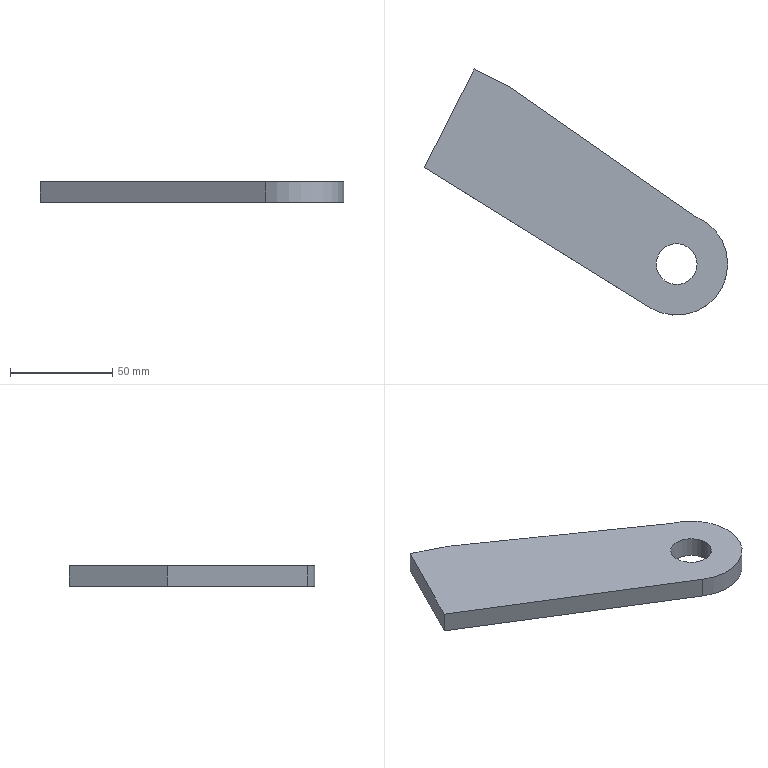Component | SolidWorks | Part15-1 | 1 solid | 9 faces | box 148.59 x 120.54 x 10 mm | volume 76558 mm3 | plane 6 | cylinder 3 | commonest cylinder face diameters 20 x2 50 x1
STEP:
#1=COLOUR_RGB('',0.7922,0.8196,0.9333);
#2=FILL_AREA_STYLE_COLOUR('',#1);
#3=FILL_AREA_STYLE('',(#2));
#4=SURFACE_STYLE_FILL_AREA(#3);
#5=SURFACE_SIDE_STYLE('',(#4));
#6=SURFACE_STYLE_USAGE(.BOTH.,#5);
#7=PRESENTATION_STYLE_ASSIGNMENT((#6));
#8=CARTESIAN_POINT('',(16.56,-46.225,83.582));
#9=VERTEX_POINT('',#8);
#10=CARTESIAN_POINT('',(17.262,-46.581,83.582));
#11=VERTEX_POINT('',#10);
#12=CARTESIAN_POINT('',(16.911,-46.403,83.582));
#13=DIRECTION('',(-0.,-0.,1.));
#14=DIRECTION('',(0.892,-0.4521,-0.));
#15=AXIS2_PLACEMENT_3D('',#12,#13,#14);
#16=CIRCLE('',#15,0.3937);
#17=EDGE_CURVE('',#9,#11,#16,.T.);
#18=ORIENTED_EDGE('',*,*,#17,.T.);
#19=CARTESIAN_POINT('',(17.262,-46.581,83.188));
#20=VERTEX_POINT('',#19);
#21=CARTESIAN_POINT('',(17.262,-46.581,83.582));
#22=DIRECTION('',(0.,0.,-1.));
#23=VECTOR('',#22,39.37);
#24=LINE('',#21,#23);
#25=EDGE_CURVE('',#11,#20,#24,.T.);
#26=ORIENTED_EDGE('',*,*,#25,.T.);
#27=CARTESIAN_POINT('',(16.56,-46.225,83.188));
#28=VERTEX_POINT('',#27);
#29=CARTESIAN_POINT('',(16.911,-46.403,83.188));
#30=DIRECTION('',(-0.,-0.,1.));
#31=DIRECTION('',(0.892,-0.4521,-0.));
#32=AXIS2_PLACEMENT_3D('',#29,#30,#31);
#33=CIRCLE('',#32,0.3937);
#34=EDGE_CURVE('',#28,#20,#33,.T.);
#35=ORIENTED_EDGE('',*,*,#34,.F.);
#36=CARTESIAN_POINT('',(16.56,-46.225,83.582));
#37=DIRECTION('',(0.,0.,-1.));
#38=VECTOR('',#37,39.37);
#39=LINE('',#36,#38);
#40=EDGE_CURVE('',#9,#28,#39,.T.);
#41=ORIENTED_EDGE('',*,*,#40,.F.);
#42=EDGE_LOOP('',(#18,#26,#35,#41));
#43=FACE_OUTER_BOUND('',#42,.T.);
#44=CARTESIAN_POINT('',(16.911,-46.403,83.582));
#45=DIRECTION('',(0.,0.,-1.));
#46=DIRECTION('',(-0.892,0.4521,0.));
#47=AXIS2_PLACEMENT_3D('',#44,#45,#46);
#48=CYLINDRICAL_SURFACE('',#47,0.3937);
#49=ADVANCED_FACE('',(#43),#48,.F.);
#50=CARTESIAN_POINT('',(12.045,-44.54,83.188));
#51=VERTEX_POINT('',#50);
#52=CARTESIAN_POINT('',(16.393,-47.24,83.188));
#53=VERTEX_POINT('',#52);
#54=CARTESIAN_POINT('',(13.395,-45.378,83.188));
#55=DIRECTION('',(0.8495,-0.5275,-0.));
#56=VECTOR('',#55,39.37);
#57=LINE('',#54,#56);
#58=EDGE_CURVE('',#51,#53,#57,.T.);
#59=ORIENTED_EDGE('',*,*,#58,.T.);
#60=CARTESIAN_POINT('',(16.393,-47.24,83.582));
#61=VERTEX_POINT('',#60);
#62=CARTESIAN_POINT('',(16.393,-47.24,83.582));
#63=DIRECTION('',(0.,0.,-1.));
#64=VECTOR('',#63,39.37);
#65=LINE('',#62,#64);
#66=EDGE_CURVE('',#61,#53,#65,.T.);
#67=ORIENTED_EDGE('',*,*,#66,.F.);
#68=CARTESIAN_POINT('',(12.045,-44.54,83.582));
#69=VERTEX_POINT('',#68);
#70=CARTESIAN_POINT('',(13.395,-45.378,83.582));
#71=DIRECTION('',(0.8495,-0.5275,-0.));
#72=VECTOR('',#71,39.37);
#73=LINE('',#70,#72);
#74=EDGE_CURVE('',#69,#61,#73,.T.);
#75=ORIENTED_EDGE('',*,*,#74,.F.);
#76=CARTESIAN_POINT('',(12.045,-44.54,83.582));
#77=DIRECTION('',(0.,0.,-1.));
#78=VECTOR('',#77,39.37);
#79=LINE('',#76,#78);
#80=EDGE_CURVE('',#69,#51,#79,.T.);
#81=ORIENTED_EDGE('',*,*,#80,.T.);
#82=EDGE_LOOP('',(#59,#67,#75,#81));
#83=FACE_OUTER_BOUND('',#82,.T.);
#84=CARTESIAN_POINT('',(13.395,-45.378,83.582));
#85=DIRECTION('',(0.5275,0.8495,0.));
#86=DIRECTION('',(-0.8495,0.5275,0.));
#87=AXIS2_PLACEMENT_3D('',#84,#85,#86);
#88=PLANE('',#87);
#89=ADVANCED_FACE('',(#83),#88,.F.);
#90=CARTESIAN_POINT('',(17.281,-45.491,83.188));
#91=VERTEX_POINT('',#90);
#92=CARTESIAN_POINT('',(16.911,-46.403,83.188));
#93=DIRECTION('',(-0.,-0.,1.));
#94=DIRECTION('',(0.892,-0.4521,-0.));
#95=AXIS2_PLACEMENT_3D('',#92,#93,#94);
#96=CIRCLE('',#95,0.9843);
#97=EDGE_CURVE('',#53,#91,#96,.T.);
#98=ORIENTED_EDGE('',*,*,#97,.T.);
#99=CARTESIAN_POINT('',(17.281,-45.491,83.582));
#100=VERTEX_POINT('',#99);
#101=CARTESIAN_POINT('',(17.281,-45.491,83.582));
#102=DIRECTION('',(0.,0.,-1.));
#103=VECTOR('',#102,39.37);
#104=LINE('',#101,#103);
#105=EDGE_CURVE('',#100,#91,#104,.T.);
#106=ORIENTED_EDGE('',*,*,#105,.F.);
#107=CARTESIAN_POINT('',(16.911,-46.403,83.582));
#108=DIRECTION('',(-0.,-0.,1.));
#109=DIRECTION('',(0.892,-0.4521,-0.));
#110=AXIS2_PLACEMENT_3D('',#107,#108,#109);
#111=CIRCLE('',#110,0.9843);
#112=EDGE_CURVE('',#61,#100,#111,.T.);
#113=ORIENTED_EDGE('',*,*,#112,.F.);
#114=ORIENTED_EDGE('',*,*,#66,.T.);
#115=EDGE_LOOP('',(#98,#106,#113,#114));
#116=FACE_OUTER_BOUND('',#115,.T.);
#117=CARTESIAN_POINT('',(16.911,-46.403,83.582));
#118=DIRECTION('',(0.,0.,-1.));
#119=DIRECTION('',(-0.892,0.4521,0.));
#120=AXIS2_PLACEMENT_3D('',#117,#118,#119);
#121=CYLINDRICAL_SURFACE('',#120,0.9843);
#122=ADVANCED_FACE('',(#116),#121,.T.);
#123=CARTESIAN_POINT('',(13.71,-42.997,83.188));
#124=VERTEX_POINT('',#123);
#125=CARTESIAN_POINT('',(14.61,-43.626,83.188));
#126=DIRECTION('',(0.8199,-0.5725,-0.));
#127=VECTOR('',#126,39.37);
#128=LINE('',#125,#127);
#129=EDGE_CURVE('',#124,#91,#128,.T.);
#130=ORIENTED_EDGE('',*,*,#129,.F.);
#131=CARTESIAN_POINT('',(13.71,-42.997,83.582));
#132=VERTEX_POINT('',#131);
#133=CARTESIAN_POINT('',(13.71,-42.997,83.582));
#134=DIRECTION('',(0.,0.,-1.));
#135=VECTOR('',#134,39.37);
#136=LINE('',#133,#135);
#137=EDGE_CURVE('',#132,#124,#136,.T.);
#138=ORIENTED_EDGE('',*,*,#137,.F.);
#139=CARTESIAN_POINT('',(14.61,-43.626,83.582));
#140=DIRECTION('',(0.8199,-0.5725,-0.));
#141=VECTOR('',#140,39.37);
#142=LINE('',#139,#141);
#143=EDGE_CURVE('',#132,#100,#142,.T.);
#144=ORIENTED_EDGE('',*,*,#143,.T.);
#145=ORIENTED_EDGE('',*,*,#105,.T.);
#146=EDGE_LOOP('',(#130,#138,#144,#145));
#147=FACE_OUTER_BOUND('',#146,.T.);
#148=CARTESIAN_POINT('',(14.61,-43.626,83.582));
#149=DIRECTION('',(0.5725,0.8199,0.));
#150=DIRECTION('',(-0.8199,0.5725,0.));
#151=AXIS2_PLACEMENT_3D('',#148,#149,#150);
#152=PLANE('',#151);
#153=ADVANCED_FACE('',(#147),#152,.T.);
#154=CARTESIAN_POINT('',(13.007,-42.641,83.188));
#155=VERTEX_POINT('',#154);
#156=CARTESIAN_POINT('',(14.43,-43.362,83.188));
#157=DIRECTION('',(0.892,-0.4521,-0.));
#158=VECTOR('',#157,39.37);
#159=LINE('',#156,#158);
#160=EDGE_CURVE('',#155,#124,#159,.T.);
#161=ORIENTED_EDGE('',*,*,#160,.F.);
#162=CARTESIAN_POINT('',(13.007,-42.641,83.582));
#163=VERTEX_POINT('',#162);
#164=CARTESIAN_POINT('',(13.007,-42.641,83.582));
#165=DIRECTION('',(0.,0.,-1.));
#166=VECTOR('',#165,39.37);
#167=LINE('',#164,#166);
#168=EDGE_CURVE('',#163,#155,#167,.T.);
#169=ORIENTED_EDGE('',*,*,#168,.F.);
#170=CARTESIAN_POINT('',(14.43,-43.362,83.582));
#171=DIRECTION('',(0.892,-0.4521,-0.));
#172=VECTOR('',#171,39.37);
#173=LINE('',#170,#172);
#174=EDGE_CURVE('',#163,#132,#173,.T.);
#175=ORIENTED_EDGE('',*,*,#174,.T.);
#176=ORIENTED_EDGE('',*,*,#137,.T.);
#177=EDGE_LOOP('',(#161,#169,#175,#176));
#178=FACE_OUTER_BOUND('',#177,.T.);
#179=CARTESIAN_POINT('',(14.43,-43.362,83.582));
#180=DIRECTION('',(0.4521,0.892,0.));
#181=DIRECTION('',(-0.,-0.,1.));
#182=AXIS2_PLACEMENT_3D('',#179,#180,#181);
#183=PLANE('',#182);
#184=ADVANCED_FACE('',(#178),#183,.T.);
#185=CARTESIAN_POINT('',(12.045,-44.54,83.188));
#186=DIRECTION('',(0.4521,0.892,0.));
#187=VECTOR('',#186,39.37);
#188=LINE('',#185,#187);
#189=EDGE_CURVE('',#51,#155,#188,.T.);
#190=ORIENTED_EDGE('',*,*,#189,.F.);
#191=ORIENTED_EDGE('',*,*,#80,.F.);
#192=CARTESIAN_POINT('',(12.045,-44.54,83.582));
#193=DIRECTION('',(0.4521,0.892,0.));
#194=VECTOR('',#193,39.37);
#195=LINE('',#192,#194);
#196=EDGE_CURVE('',#69,#163,#195,.T.);
#197=ORIENTED_EDGE('',*,*,#196,.T.);
#198=ORIENTED_EDGE('',*,*,#168,.T.);
#199=EDGE_LOOP('',(#190,#191,#197,#198));
#200=FACE_OUTER_BOUND('',#199,.T.);
#201=CARTESIAN_POINT('',(12.045,-44.54,83.582));
#202=DIRECTION('',(-0.892,0.4521,0.));
#203=DIRECTION('',(-0.,-0.,1.));
#204=AXIS2_PLACEMENT_3D('',#201,#202,#203);
#205=PLANE('',#204);
#206=ADVANCED_FACE('',(#200),#205,.T.);
#207=ORIENTED_EDGE('',*,*,#25,.F.);
#208=CARTESIAN_POINT('',(16.911,-46.403,83.582));
#209=DIRECTION('',(-0.,-0.,1.));
#210=DIRECTION('',(0.892,-0.4521,-0.));
#211=AXIS2_PLACEMENT_3D('',#208,#209,#210);
#212=CIRCLE('',#211,0.3937);
#213=EDGE_CURVE('',#11,#9,#212,.T.);
#214=ORIENTED_EDGE('',*,*,#213,.T.);
#215=ORIENTED_EDGE('',*,*,#40,.T.);
#216=CARTESIAN_POINT('',(16.911,-46.403,83.188));
#217=DIRECTION('',(-0.,-0.,1.));
#218=DIRECTION('',(0.892,-0.4521,-0.));
#219=AXIS2_PLACEMENT_3D('',#216,#217,#218);
#220=CIRCLE('',#219,0.3937);
#221=EDGE_CURVE('',#20,#28,#220,.T.);
#222=ORIENTED_EDGE('',*,*,#221,.F.);
#223=EDGE_LOOP('',(#207,#214,#215,#222));
#224=FACE_OUTER_BOUND('',#223,.T.);
#225=CARTESIAN_POINT('',(16.911,-46.403,83.582));
#226=DIRECTION('',(0.,0.,-1.));
#227=DIRECTION('',(-0.892,0.4521,0.));
#228=AXIS2_PLACEMENT_3D('',#225,#226,#227);
#229=CYLINDRICAL_SURFACE('',#228,0.3937);
#230=ADVANCED_FACE('',(#224),#229,.F.);
#231=ORIENTED_EDGE('',*,*,#74,.T.);
#232=ORIENTED_EDGE('',*,*,#112,.T.);
#233=ORIENTED_EDGE('',*,*,#143,.F.);
#234=ORIENTED_EDGE('',*,*,#174,.F.);
#235=ORIENTED_EDGE('',*,*,#196,.F.);
#236=EDGE_LOOP('',(#231,#232,#233,#234,#235));
#237=FACE_OUTER_BOUND('',#236,.T.);
#238=ORIENTED_EDGE('',*,*,#17,.F.);
#239=ORIENTED_EDGE('',*,*,#213,.F.);
#240=EDGE_LOOP('',(#238,#239));
#241=FACE_BOUND('',#240,.T.);
#242=CARTESIAN_POINT('',(13.468,-45.261,83.582));
#243=DIRECTION('',(-0.,-0.,1.));
#244=DIRECTION('',(0.892,-0.4521,-0.));
#245=AXIS2_PLACEMENT_3D('',#242,#243,#244);
#246=PLANE('',#245);
#247=ADVANCED_FACE('',(#237,#241),#246,.T.);
#248=ORIENTED_EDGE('',*,*,#58,.F.);
#249=ORIENTED_EDGE('',*,*,#189,.T.);
#250=ORIENTED_EDGE('',*,*,#160,.T.);
#251=ORIENTED_EDGE('',*,*,#129,.T.);
#252=ORIENTED_EDGE('',*,*,#97,.F.);
#253=EDGE_LOOP('',(#248,#249,#250,#251,#252));
#254=FACE_OUTER_BOUND('',#253,.T.);
#255=ORIENTED_EDGE('',*,*,#34,.T.);
#256=ORIENTED_EDGE('',*,*,#221,.T.);
#257=EDGE_LOOP('',(#255,#256));
#258=FACE_BOUND('',#257,.T.);
#259=CARTESIAN_POINT('',(13.468,-45.261,83.188));
#260=DIRECTION('',(-0.,-0.,1.));
#261=DIRECTION('',(0.892,-0.4521,-0.));
#262=AXIS2_PLACEMENT_3D('',#259,#260,#261);
#263=PLANE('',#262);
#264=ADVANCED_FACE('',(#254,#258),#263,.F.);
#265=CLOSED_SHELL('',(#49,#89,#122,#153,#184,#206,#230,#247,#264));
#266=MANIFOLD_SOLID_BREP('',#265);
#267=STYLED_ITEM('',(#7),#266);
#268=PRESENTATION_LAYER_ASSIGNMENT('','',(#267));
#269=(LENGTH_UNIT()NAMED_UNIT(*)SI_UNIT($,.METRE.));
#270=LENGTH_MEASURE_WITH_UNIT(LENGTH_MEASURE(0.0254),#269);
#271=DIMENSIONAL_EXPONENTS(1.,0.,0.,0.,0.,0.,0.);
#272=(CONVERSION_BASED_UNIT('',#270)LENGTH_UNIT()NAMED_UNIT(#271));
#273=UNCERTAINTY_MEASURE_WITH_UNIT(LENGTH_MEASURE(0.00001),#272,'','');
#274=(NAMED_UNIT(*)PLANE_ANGLE_UNIT()SI_UNIT($,.RADIAN.));
#275=(NAMED_UNIT(*)SI_UNIT($,.STERADIAN.)SOLID_ANGLE_UNIT());
#276=(GEOMETRIC_REPRESENTATION_CONTEXT(3)GLOBAL_UNCERTAINTY_ASSIGNED_CONTEXT((#273))GLOBAL_UNIT_ASSIGNED_CONTEXT((#272,#274,#275))REPRESENTATION_CONTEXT('',''));
#277=MECHANICAL_DESIGN_GEOMETRIC_PRESENTATION_REPRESENTATION('',(#267),#276);
#278=CARTESIAN_POINT('',(0.,0.,0.));
#279=DIRECTION('',(0.,0.,1.));
#280=DIRECTION('',(1.,0.,0.));
#281=AXIS2_PLACEMENT_3D('',#278,#279,#280);
#282=(LENGTH_UNIT()NAMED_UNIT(*)SI_UNIT($,.METRE.));
#283=LENGTH_MEASURE_WITH_UNIT(LENGTH_MEASURE(0.0254),#282);
#284=DIMENSIONAL_EXPONENTS(1.,0.,0.,0.,0.,0.,0.);
#285=(CONVERSION_BASED_UNIT('',#283)LENGTH_UNIT()NAMED_UNIT(#284));
#286=UNCERTAINTY_MEASURE_WITH_UNIT(LENGTH_MEASURE(0.00001),#285,'','');
#287=(NAMED_UNIT(*)PLANE_ANGLE_UNIT()SI_UNIT($,.RADIAN.));
#288=(NAMED_UNIT(*)SI_UNIT($,.STERADIAN.)SOLID_ANGLE_UNIT());
#289=(GEOMETRIC_REPRESENTATION_CONTEXT(3)GLOBAL_UNCERTAINTY_ASSIGNED_CONTEXT((#286))GLOBAL_UNIT_ASSIGNED_CONTEXT((#285,#287,#288))REPRESENTATION_CONTEXT('',''));
#290=ADVANCED_BREP_SHAPE_REPRESENTATION('',(#266,#281),#289);